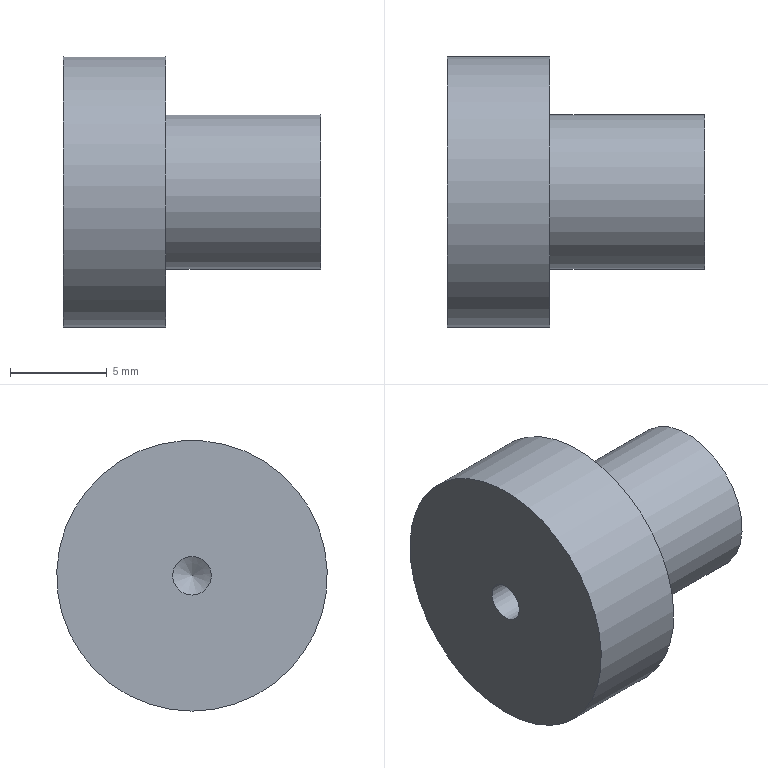Component | NX | SPRING_SEAT | 1 solid | 7 faces | box 13.3 x 14 x 14 mm | volume 1202 mm3 | cylinder 3 | plane 3 | cone 1 | commonest cylinder face diameters 14 x1 8 x1 2 x1
STEP:
#1=CARTESIAN_POINT('',(0.,0.,0.));
#2=DIRECTION('',(0.,0.,1.));
#3=DIRECTION('',(1.,0.,0.));
#4=AXIS2_PLACEMENT_3D('',#1,#2,#3);
#5=CARTESIAN_POINT('',(9.99,-0.,13.));
#6=VERTEX_POINT('',#5);
#7=CARTESIAN_POINT('',(9.99,-0.,20.));
#8=DIRECTION('',(1.,0.,0.));
#9=DIRECTION('',(0.,0.,-1.));
#10=AXIS2_PLACEMENT_3D('',#7,#8,#9);
#11=CIRCLE('',#10,7.);
#12=CARTESIAN_POINT('',(9.99,-0.,20.));
#13=DIRECTION('',(-1.,0.,0.));
#14=DIRECTION('',(0.,0.,1.));
#15=AXIS2_PLACEMENT_3D('',#12,#13,#14);
#16=CYLINDRICAL_SURFACE('',#15,7.);
#17=CARTESIAN_POINT('',(9.425,0.));
#18=DIRECTION('',(-1.,0.));
#19=VECTOR('',#18,1.);
#20=LINE('',#17,#19);
#21=(GEOMETRIC_REPRESENTATION_CONTEXT(2)PARAMETRIC_REPRESENTATION_CONTEXT()REPRESENTATION_CONTEXT('',''));
#22=DEFINITIONAL_REPRESENTATION('',(#20),#21);
#23=PCURVE('',#16,#22);
#24=CARTESIAN_POINT('',(9.99,-0.,20.));
#25=DIRECTION('',(1.,0.,0.));
#26=DIRECTION('',(0.,0.,-1.));
#27=AXIS2_PLACEMENT_3D('',#24,#25,#26);
#28=PLANE('',#27);
#29=CARTESIAN_POINT('',(0.,0.));
#30=DIRECTION('',(1.,0.));
#31=AXIS2_PLACEMENT_2D('',#29,#30);
#32=CIRCLE('',#31,7.);
#33=(GEOMETRIC_REPRESENTATION_CONTEXT(2)PARAMETRIC_REPRESENTATION_CONTEXT()REPRESENTATION_CONTEXT('',''));
#34=DEFINITIONAL_REPRESENTATION('',(#32),#33);
#35=PCURVE('',#28,#34);
#36=SURFACE_CURVE('',#11,(#23,#35),.PCURVE_S1.);
#37=EDGE_CURVE('',#6,#6,#36,.T.);
#38=ORIENTED_EDGE('',*,*,#37,.F.);
#39=CARTESIAN_POINT('',(4.69,-0.,13.));
#40=VERTEX_POINT('',#39);
#41=CARTESIAN_POINT('',(9.99,-0.,13.));
#42=CARTESIAN_POINT('',(4.69,-0.,13.));
#43=B_SPLINE_CURVE_WITH_KNOTS('',1,(#41,#42),.UNSPECIFIED.,.F.,.F.,(2,2),(0.,5.3),.PIECEWISE_BEZIER_KNOTS.);
#44=CARTESIAN_POINT('',(9.425,0.));
#45=DIRECTION('',(0.,1.));
#46=VECTOR('',#45,1.);
#47=LINE('',#44,#46);
#48=(GEOMETRIC_REPRESENTATION_CONTEXT(2)PARAMETRIC_REPRESENTATION_CONTEXT()REPRESENTATION_CONTEXT('',''));
#49=DEFINITIONAL_REPRESENTATION('',(#47),#48);
#50=PCURVE('',#16,#49);
#51=CARTESIAN_POINT('',(3.142,0.));
#52=DIRECTION('',(0.,1.));
#53=VECTOR('',#52,1.);
#54=LINE('',#51,#53);
#55=(GEOMETRIC_REPRESENTATION_CONTEXT(2)PARAMETRIC_REPRESENTATION_CONTEXT()REPRESENTATION_CONTEXT('',''));
#56=DEFINITIONAL_REPRESENTATION('',(#54),#55);
#57=PCURVE('',#16,#56);
#58=SEAM_CURVE('',#43,(#50,#57),.PCURVE_S1.);
#59=EDGE_CURVE('',#6,#40,#58,.T.);
#60=ORIENTED_EDGE('',*,*,#59,.T.);
#61=CARTESIAN_POINT('',(4.69,-0.,20.));
#62=DIRECTION('',(1.,0.,0.));
#63=DIRECTION('',(0.,0.,-1.));
#64=AXIS2_PLACEMENT_3D('',#61,#62,#63);
#65=CIRCLE('',#64,7.);
#66=CARTESIAN_POINT('',(9.425,5.3));
#67=DIRECTION('',(-1.,0.));
#68=VECTOR('',#67,1.);
#69=LINE('',#66,#68);
#70=(GEOMETRIC_REPRESENTATION_CONTEXT(2)PARAMETRIC_REPRESENTATION_CONTEXT()REPRESENTATION_CONTEXT('',''));
#71=DEFINITIONAL_REPRESENTATION('',(#69),#70);
#72=PCURVE('',#16,#71);
#73=CARTESIAN_POINT('',(4.69,-0.,20.));
#74=DIRECTION('',(1.,0.,0.));
#75=DIRECTION('',(0.,0.,-1.));
#76=AXIS2_PLACEMENT_3D('',#73,#74,#75);
#77=PLANE('',#76);
#78=CARTESIAN_POINT('',(0.,0.));
#79=DIRECTION('',(1.,0.));
#80=AXIS2_PLACEMENT_2D('',#78,#79);
#81=CIRCLE('',#80,7.);
#82=(GEOMETRIC_REPRESENTATION_CONTEXT(2)PARAMETRIC_REPRESENTATION_CONTEXT()REPRESENTATION_CONTEXT('',''));
#83=DEFINITIONAL_REPRESENTATION('',(#81),#82);
#84=PCURVE('',#77,#83);
#85=SURFACE_CURVE('',#65,(#72,#84),.PCURVE_S1.);
#86=EDGE_CURVE('',#40,#40,#85,.T.);
#87=ORIENTED_EDGE('',*,*,#86,.T.);
#88=ORIENTED_EDGE('',*,*,#59,.F.);
#89=EDGE_LOOP('',(#38,#60,#87,#88));
#90=FACE_BOUND('',#89,.T.);
#91=ADVANCED_FACE('',(#90),#16,.T.);
#92=CARTESIAN_POINT('',(9.99,-0.,16.));
#93=VERTEX_POINT('',#92);
#94=CARTESIAN_POINT('',(9.99,-0.,20.));
#95=DIRECTION('',(1.,0.,0.));
#96=DIRECTION('',(0.,0.,-1.));
#97=AXIS2_PLACEMENT_3D('',#94,#95,#96);
#98=CIRCLE('',#97,4.);
#99=CARTESIAN_POINT('',(0.,0.));
#100=DIRECTION('',(1.,0.));
#101=AXIS2_PLACEMENT_2D('',#99,#100);
#102=CIRCLE('',#101,4.);
#103=(GEOMETRIC_REPRESENTATION_CONTEXT(2)PARAMETRIC_REPRESENTATION_CONTEXT()REPRESENTATION_CONTEXT('',''));
#104=DEFINITIONAL_REPRESENTATION('',(#102),#103);
#105=PCURVE('',#28,#104);
#106=CARTESIAN_POINT('',(17.99,-0.,20.));
#107=DIRECTION('',(-1.,0.,0.));
#108=DIRECTION('',(0.,0.,1.));
#109=AXIS2_PLACEMENT_3D('',#106,#107,#108);
#110=CYLINDRICAL_SURFACE('',#109,4.);
#111=CARTESIAN_POINT('',(9.425,8.));
#112=DIRECTION('',(-1.,0.));
#113=VECTOR('',#112,1.);
#114=LINE('',#111,#113);
#115=(GEOMETRIC_REPRESENTATION_CONTEXT(2)PARAMETRIC_REPRESENTATION_CONTEXT()REPRESENTATION_CONTEXT('',''));
#116=DEFINITIONAL_REPRESENTATION('',(#114),#115);
#117=PCURVE('',#110,#116);
#118=SURFACE_CURVE('',#98,(#105,#117),.PCURVE_S1.);
#119=EDGE_CURVE('',#93,#93,#118,.T.);
#120=ORIENTED_EDGE('',*,*,#119,.F.);
#121=EDGE_LOOP('',(#120));
#122=FACE_BOUND('',#121,.T.);
#123=ORIENTED_EDGE('',*,*,#37,.T.);
#124=EDGE_LOOP('',(#123));
#125=FACE_BOUND('',#124,.T.);
#126=ADVANCED_FACE('',(#122,#125),#28,.T.);
#127=CARTESIAN_POINT('',(4.69,-0.,19.));
#128=VERTEX_POINT('',#127);
#129=CARTESIAN_POINT('',(4.69,-0.,20.));
#130=DIRECTION('',(1.,0.,0.));
#131=DIRECTION('',(0.,0.,-1.));
#132=AXIS2_PLACEMENT_3D('',#129,#130,#131);
#133=CIRCLE('',#132,1.);
#134=CARTESIAN_POINT('',(0.,0.));
#135=DIRECTION('',(1.,0.));
#136=AXIS2_PLACEMENT_2D('',#134,#135);
#137=CIRCLE('',#136,1.);
#138=(GEOMETRIC_REPRESENTATION_CONTEXT(2)PARAMETRIC_REPRESENTATION_CONTEXT()REPRESENTATION_CONTEXT('',''));
#139=DEFINITIONAL_REPRESENTATION('',(#137),#138);
#140=PCURVE('',#77,#139);
#141=CARTESIAN_POINT('',(4.69,-0.,20.));
#142=DIRECTION('',(1.,0.,0.));
#143=DIRECTION('',(0.,0.,-1.));
#144=AXIS2_PLACEMENT_3D('',#141,#142,#143);
#145=CYLINDRICAL_SURFACE('',#144,1.);
#146=CARTESIAN_POINT('',(0.,0.));
#147=DIRECTION('',(1.,0.));
#148=VECTOR('',#147,1.);
#149=LINE('',#146,#148);
#150=(GEOMETRIC_REPRESENTATION_CONTEXT(2)PARAMETRIC_REPRESENTATION_CONTEXT()REPRESENTATION_CONTEXT('',''));
#151=DEFINITIONAL_REPRESENTATION('',(#149),#150);
#152=PCURVE('',#145,#151);
#153=SURFACE_CURVE('',#133,(#140,#152),.PCURVE_S1.);
#154=EDGE_CURVE('',#128,#128,#153,.T.);
#155=ORIENTED_EDGE('',*,*,#154,.T.);
#156=EDGE_LOOP('',(#155));
#157=FACE_BOUND('',#156,.T.);
#158=ORIENTED_EDGE('',*,*,#86,.F.);
#159=EDGE_LOOP('',(#158));
#160=FACE_BOUND('',#159,.T.);
#161=ADVANCED_FACE('',(#157,#160),#77,.F.);
#162=CARTESIAN_POINT('',(17.99,-0.,16.));
#163=VERTEX_POINT('',#162);
#164=CARTESIAN_POINT('',(17.99,-0.,20.));
#165=DIRECTION('',(1.,0.,0.));
#166=DIRECTION('',(0.,0.,-1.));
#167=AXIS2_PLACEMENT_3D('',#164,#165,#166);
#168=CIRCLE('',#167,4.);
#169=CARTESIAN_POINT('',(9.425,0.));
#170=DIRECTION('',(-1.,0.));
#171=VECTOR('',#170,1.);
#172=LINE('',#169,#171);
#173=(GEOMETRIC_REPRESENTATION_CONTEXT(2)PARAMETRIC_REPRESENTATION_CONTEXT()REPRESENTATION_CONTEXT('',''));
#174=DEFINITIONAL_REPRESENTATION('',(#172),#173);
#175=PCURVE('',#110,#174);
#176=CARTESIAN_POINT('',(17.99,-0.,20.));
#177=DIRECTION('',(1.,0.,0.));
#178=DIRECTION('',(0.,0.,-1.));
#179=AXIS2_PLACEMENT_3D('',#176,#177,#178);
#180=PLANE('',#179);
#181=CARTESIAN_POINT('',(0.,0.));
#182=DIRECTION('',(1.,0.));
#183=AXIS2_PLACEMENT_2D('',#181,#182);
#184=CIRCLE('',#183,4.);
#185=(GEOMETRIC_REPRESENTATION_CONTEXT(2)PARAMETRIC_REPRESENTATION_CONTEXT()REPRESENTATION_CONTEXT('',''));
#186=DEFINITIONAL_REPRESENTATION('',(#184),#185);
#187=PCURVE('',#180,#186);
#188=SURFACE_CURVE('',#168,(#175,#187),.PCURVE_S1.);
#189=EDGE_CURVE('',#163,#163,#188,.T.);
#190=ORIENTED_EDGE('',*,*,#189,.F.);
#191=CARTESIAN_POINT('',(17.99,-0.,16.));
#192=CARTESIAN_POINT('',(9.99,-0.,16.));
#193=B_SPLINE_CURVE_WITH_KNOTS('',1,(#191,#192),.UNSPECIFIED.,.F.,.F.,(2,2),(0.,8.),.PIECEWISE_BEZIER_KNOTS.);
#194=CARTESIAN_POINT('',(9.425,0.));
#195=DIRECTION('',(0.,1.));
#196=VECTOR('',#195,1.);
#197=LINE('',#194,#196);
#198=(GEOMETRIC_REPRESENTATION_CONTEXT(2)PARAMETRIC_REPRESENTATION_CONTEXT()REPRESENTATION_CONTEXT('',''));
#199=DEFINITIONAL_REPRESENTATION('',(#197),#198);
#200=PCURVE('',#110,#199);
#201=CARTESIAN_POINT('',(3.142,0.));
#202=DIRECTION('',(0.,1.));
#203=VECTOR('',#202,1.);
#204=LINE('',#201,#203);
#205=(GEOMETRIC_REPRESENTATION_CONTEXT(2)PARAMETRIC_REPRESENTATION_CONTEXT()REPRESENTATION_CONTEXT('',''));
#206=DEFINITIONAL_REPRESENTATION('',(#204),#205);
#207=PCURVE('',#110,#206);
#208=SEAM_CURVE('',#193,(#200,#207),.PCURVE_S1.);
#209=EDGE_CURVE('',#163,#93,#208,.T.);
#210=ORIENTED_EDGE('',*,*,#209,.T.);
#211=ORIENTED_EDGE('',*,*,#119,.T.);
#212=ORIENTED_EDGE('',*,*,#209,.F.);
#213=EDGE_LOOP('',(#190,#210,#211,#212));
#214=FACE_BOUND('',#213,.T.);
#215=ADVANCED_FACE('',(#214),#110,.T.);
#216=ORIENTED_EDGE('',*,*,#189,.T.);
#217=EDGE_LOOP('',(#216));
#218=FACE_BOUND('',#217,.T.);
#219=ADVANCED_FACE('',(#218),#180,.T.);
#220=CARTESIAN_POINT('',(9.69,-0.,21.));
#221=VERTEX_POINT('',#220);
#222=CARTESIAN_POINT('',(9.69,-0.,19.));
#223=VERTEX_POINT('',#222);
#224=CARTESIAN_POINT('',(9.69,-0.,20.));
#225=DIRECTION('',(-1.,0.,0.));
#226=DIRECTION('',(0.,0.,-1.));
#227=AXIS2_PLACEMENT_3D('',#224,#225,#226);
#228=CIRCLE('',#227,1.);
#229=CARTESIAN_POINT('',(9.69,-0.,20.));
#230=DIRECTION('',(-1.,0.,0.));
#231=DIRECTION('',(0.,0.,1.));
#232=AXIS2_PLACEMENT_3D('',#229,#230,#231);
#233=CONICAL_SURFACE('',#232,1.,1.03);
#234=CARTESIAN_POINT('',(-3.142,0.));
#235=DIRECTION('',(1.,0.));
#236=VECTOR('',#235,1.);
#237=LINE('',#234,#236);
#238=(GEOMETRIC_REPRESENTATION_CONTEXT(2)PARAMETRIC_REPRESENTATION_CONTEXT()REPRESENTATION_CONTEXT('',''));
#239=DEFINITIONAL_REPRESENTATION('',(#237),#238);
#240=PCURVE('',#233,#239);
#241=CARTESIAN_POINT('',(6.283,5.));
#242=DIRECTION('',(-1.,0.));
#243=VECTOR('',#242,1.);
#244=LINE('',#241,#243);
#245=(GEOMETRIC_REPRESENTATION_CONTEXT(2)PARAMETRIC_REPRESENTATION_CONTEXT()REPRESENTATION_CONTEXT('',''));
#246=DEFINITIONAL_REPRESENTATION('',(#244),#245);
#247=PCURVE('',#145,#246);
#248=SURFACE_CURVE('',#228,(#240,#247),.PCURVE_S1.);
#249=EDGE_CURVE('',#221,#223,#248,.T.);
#250=ORIENTED_EDGE('',*,*,#249,.F.);
#251=CARTESIAN_POINT('',(10.291,-0.,20.));
#252=VERTEX_POINT('',#251);
#253=CARTESIAN_POINT('',(10.291,-0.,20.));
#254=CARTESIAN_POINT('',(9.69,-0.,21.));
#255=B_SPLINE_CURVE_WITH_KNOTS('',1,(#253,#254),.UNSPECIFIED.,.F.,.F.,(2,2),(-1.167,0.),.PIECEWISE_BEZIER_KNOTS.);
#256=CARTESIAN_POINT('',(0.,0.));
#257=DIRECTION('',(0.,1.));
#258=VECTOR('',#257,1.);
#259=LINE('',#256,#258);
#260=(GEOMETRIC_REPRESENTATION_CONTEXT(2)PARAMETRIC_REPRESENTATION_CONTEXT()REPRESENTATION_CONTEXT('',''));
#261=DEFINITIONAL_REPRESENTATION('',(#259),#260);
#262=PCURVE('',#233,#261);
#263=CARTESIAN_POINT('',(6.283,0.));
#264=DIRECTION('',(0.,1.));
#265=VECTOR('',#264,1.);
#266=LINE('',#263,#265);
#267=(GEOMETRIC_REPRESENTATION_CONTEXT(2)PARAMETRIC_REPRESENTATION_CONTEXT()REPRESENTATION_CONTEXT('',''));
#268=DEFINITIONAL_REPRESENTATION('',(#266),#267);
#269=PCURVE('',#233,#268);
#270=SEAM_CURVE('',#255,(#262,#269),.PCURVE_S1.);
#271=EDGE_CURVE('',#252,#221,#270,.T.);
#272=ORIENTED_EDGE('',*,*,#271,.F.);
#273=ORIENTED_EDGE('',*,*,#271,.T.);
#274=CARTESIAN_POINT('',(9.69,-0.,20.));
#275=DIRECTION('',(-1.,0.,0.));
#276=DIRECTION('',(0.,0.,-1.));
#277=AXIS2_PLACEMENT_3D('',#274,#275,#276);
#278=CIRCLE('',#277,1.);
#279=CARTESIAN_POINT('',(3.142,0.));
#280=DIRECTION('',(1.,0.));
#281=VECTOR('',#280,1.);
#282=LINE('',#279,#281);
#283=(GEOMETRIC_REPRESENTATION_CONTEXT(2)PARAMETRIC_REPRESENTATION_CONTEXT()REPRESENTATION_CONTEXT('',''));
#284=DEFINITIONAL_REPRESENTATION('',(#282),#283);
#285=PCURVE('',#233,#284);
#286=CARTESIAN_POINT('',(6.283,5.));
#287=DIRECTION('',(-1.,0.));
#288=VECTOR('',#287,1.);
#289=LINE('',#286,#288);
#290=(GEOMETRIC_REPRESENTATION_CONTEXT(2)PARAMETRIC_REPRESENTATION_CONTEXT()REPRESENTATION_CONTEXT('',''));
#291=DEFINITIONAL_REPRESENTATION('',(#289),#290);
#292=PCURVE('',#145,#291);
#293=SURFACE_CURVE('',#278,(#285,#292),.PCURVE_S1.);
#294=EDGE_CURVE('',#223,#221,#293,.T.);
#295=ORIENTED_EDGE('',*,*,#294,.F.);
#296=EDGE_LOOP('',(#250,#272,#273,#295));
#297=FACE_BOUND('',#296,.F.);
#298=ADVANCED_FACE('',(#297),#233,.F.);
#299=ORIENTED_EDGE('',*,*,#249,.T.);
#300=CARTESIAN_POINT('',(4.69,-0.,19.));
#301=CARTESIAN_POINT('',(9.69,-0.,19.));
#302=B_SPLINE_CURVE_WITH_KNOTS('',1,(#300,#301),.UNSPECIFIED.,.F.,.F.,(2,2),(0.,5.),.PIECEWISE_BEZIER_KNOTS.);
#303=CARTESIAN_POINT('',(0.,0.));
#304=DIRECTION('',(0.,1.));
#305=VECTOR('',#304,1.);
#306=LINE('',#303,#305);
#307=(GEOMETRIC_REPRESENTATION_CONTEXT(2)PARAMETRIC_REPRESENTATION_CONTEXT()REPRESENTATION_CONTEXT('',''));
#308=DEFINITIONAL_REPRESENTATION('',(#306),#307);
#309=PCURVE('',#145,#308);
#310=CARTESIAN_POINT('',(6.283,0.));
#311=DIRECTION('',(0.,1.));
#312=VECTOR('',#311,1.);
#313=LINE('',#310,#312);
#314=(GEOMETRIC_REPRESENTATION_CONTEXT(2)PARAMETRIC_REPRESENTATION_CONTEXT()REPRESENTATION_CONTEXT('',''));
#315=DEFINITIONAL_REPRESENTATION('',(#313),#314);
#316=PCURVE('',#145,#315);
#317=SEAM_CURVE('',#302,(#309,#316),.PCURVE_S1.);
#318=EDGE_CURVE('',#128,#223,#317,.T.);
#319=ORIENTED_EDGE('',*,*,#318,.F.);
#320=ORIENTED_EDGE('',*,*,#154,.T.);
#321=ORIENTED_EDGE('',*,*,#318,.T.);
#322=ORIENTED_EDGE('',*,*,#294,.T.);
#323=EDGE_LOOP('',(#299,#319,#320,#321,#322));
#324=FACE_BOUND('',#323,.F.);
#325=ADVANCED_FACE('',(#324),#145,.F.);
#326=CLOSED_SHELL('',(#91,#126,#161,#215,#219,#298,#325));
#327=MANIFOLD_SOLID_BREP('',#326);
#328=(LENGTH_UNIT()NAMED_UNIT(*)SI_UNIT(.MILLI.,.METRE.));
#329=UNCERTAINTY_MEASURE_WITH_UNIT(LENGTH_MEASURE(0.00001),#328,'','');
#330=(NAMED_UNIT(*)PLANE_ANGLE_UNIT()SI_UNIT($,.RADIAN.));
#331=(NAMED_UNIT(*)SI_UNIT($,.STERADIAN.)SOLID_ANGLE_UNIT());
#332=(GEOMETRIC_REPRESENTATION_CONTEXT(3)GLOBAL_UNCERTAINTY_ASSIGNED_CONTEXT((#329))GLOBAL_UNIT_ASSIGNED_CONTEXT((#328,#330,#331))REPRESENTATION_CONTEXT('',''));
#333=ADVANCED_BREP_SHAPE_REPRESENTATION('',(#4,#327),#332);